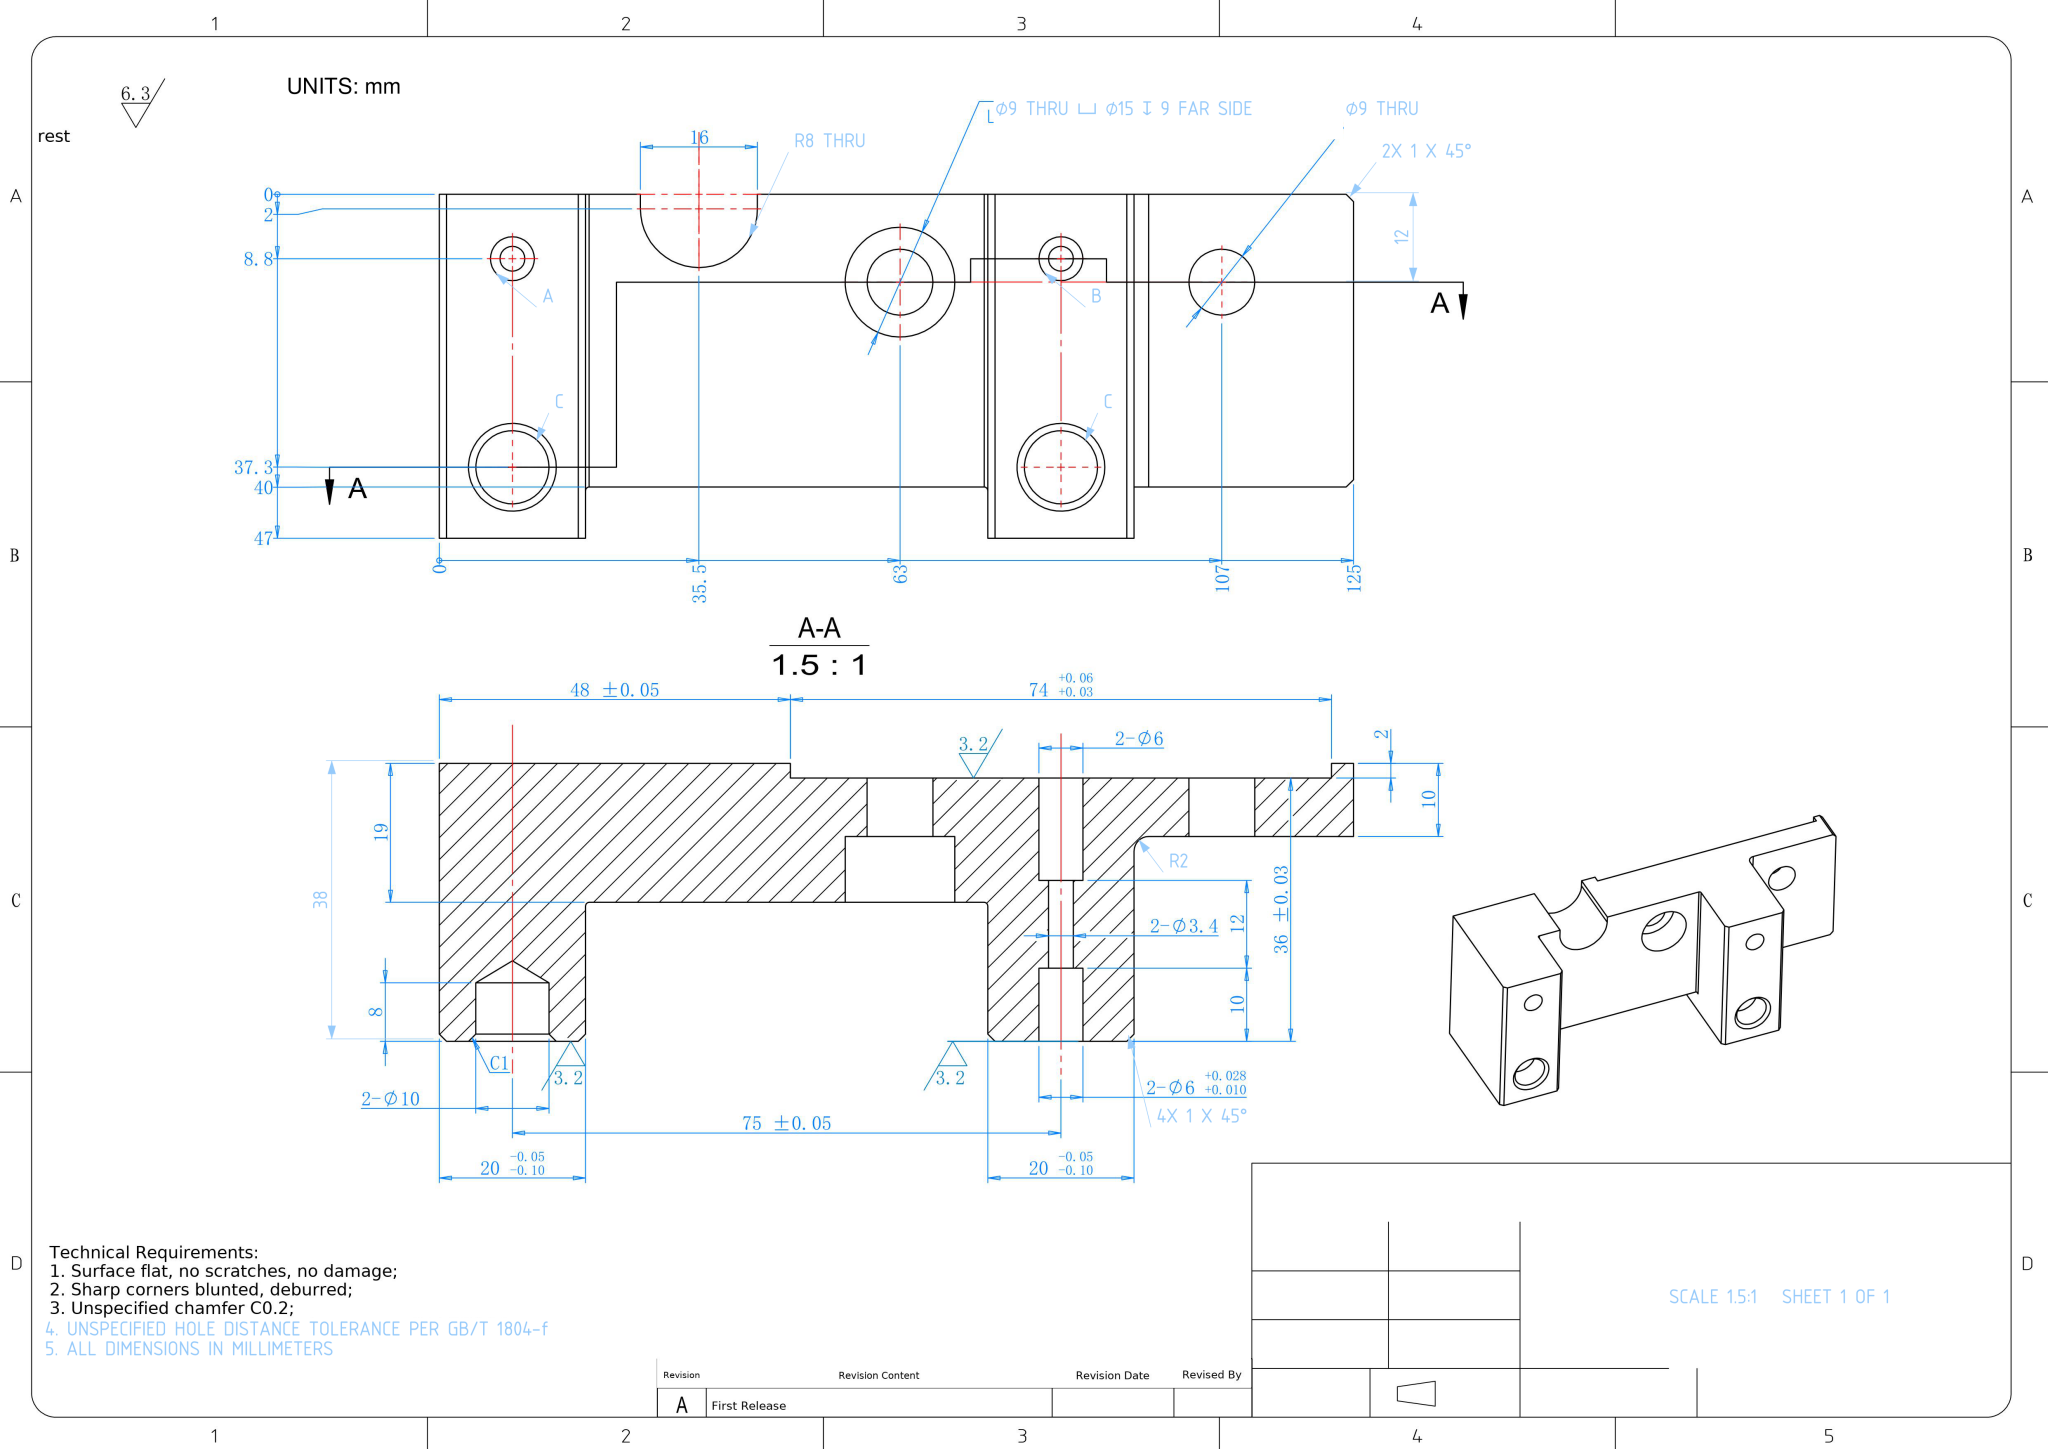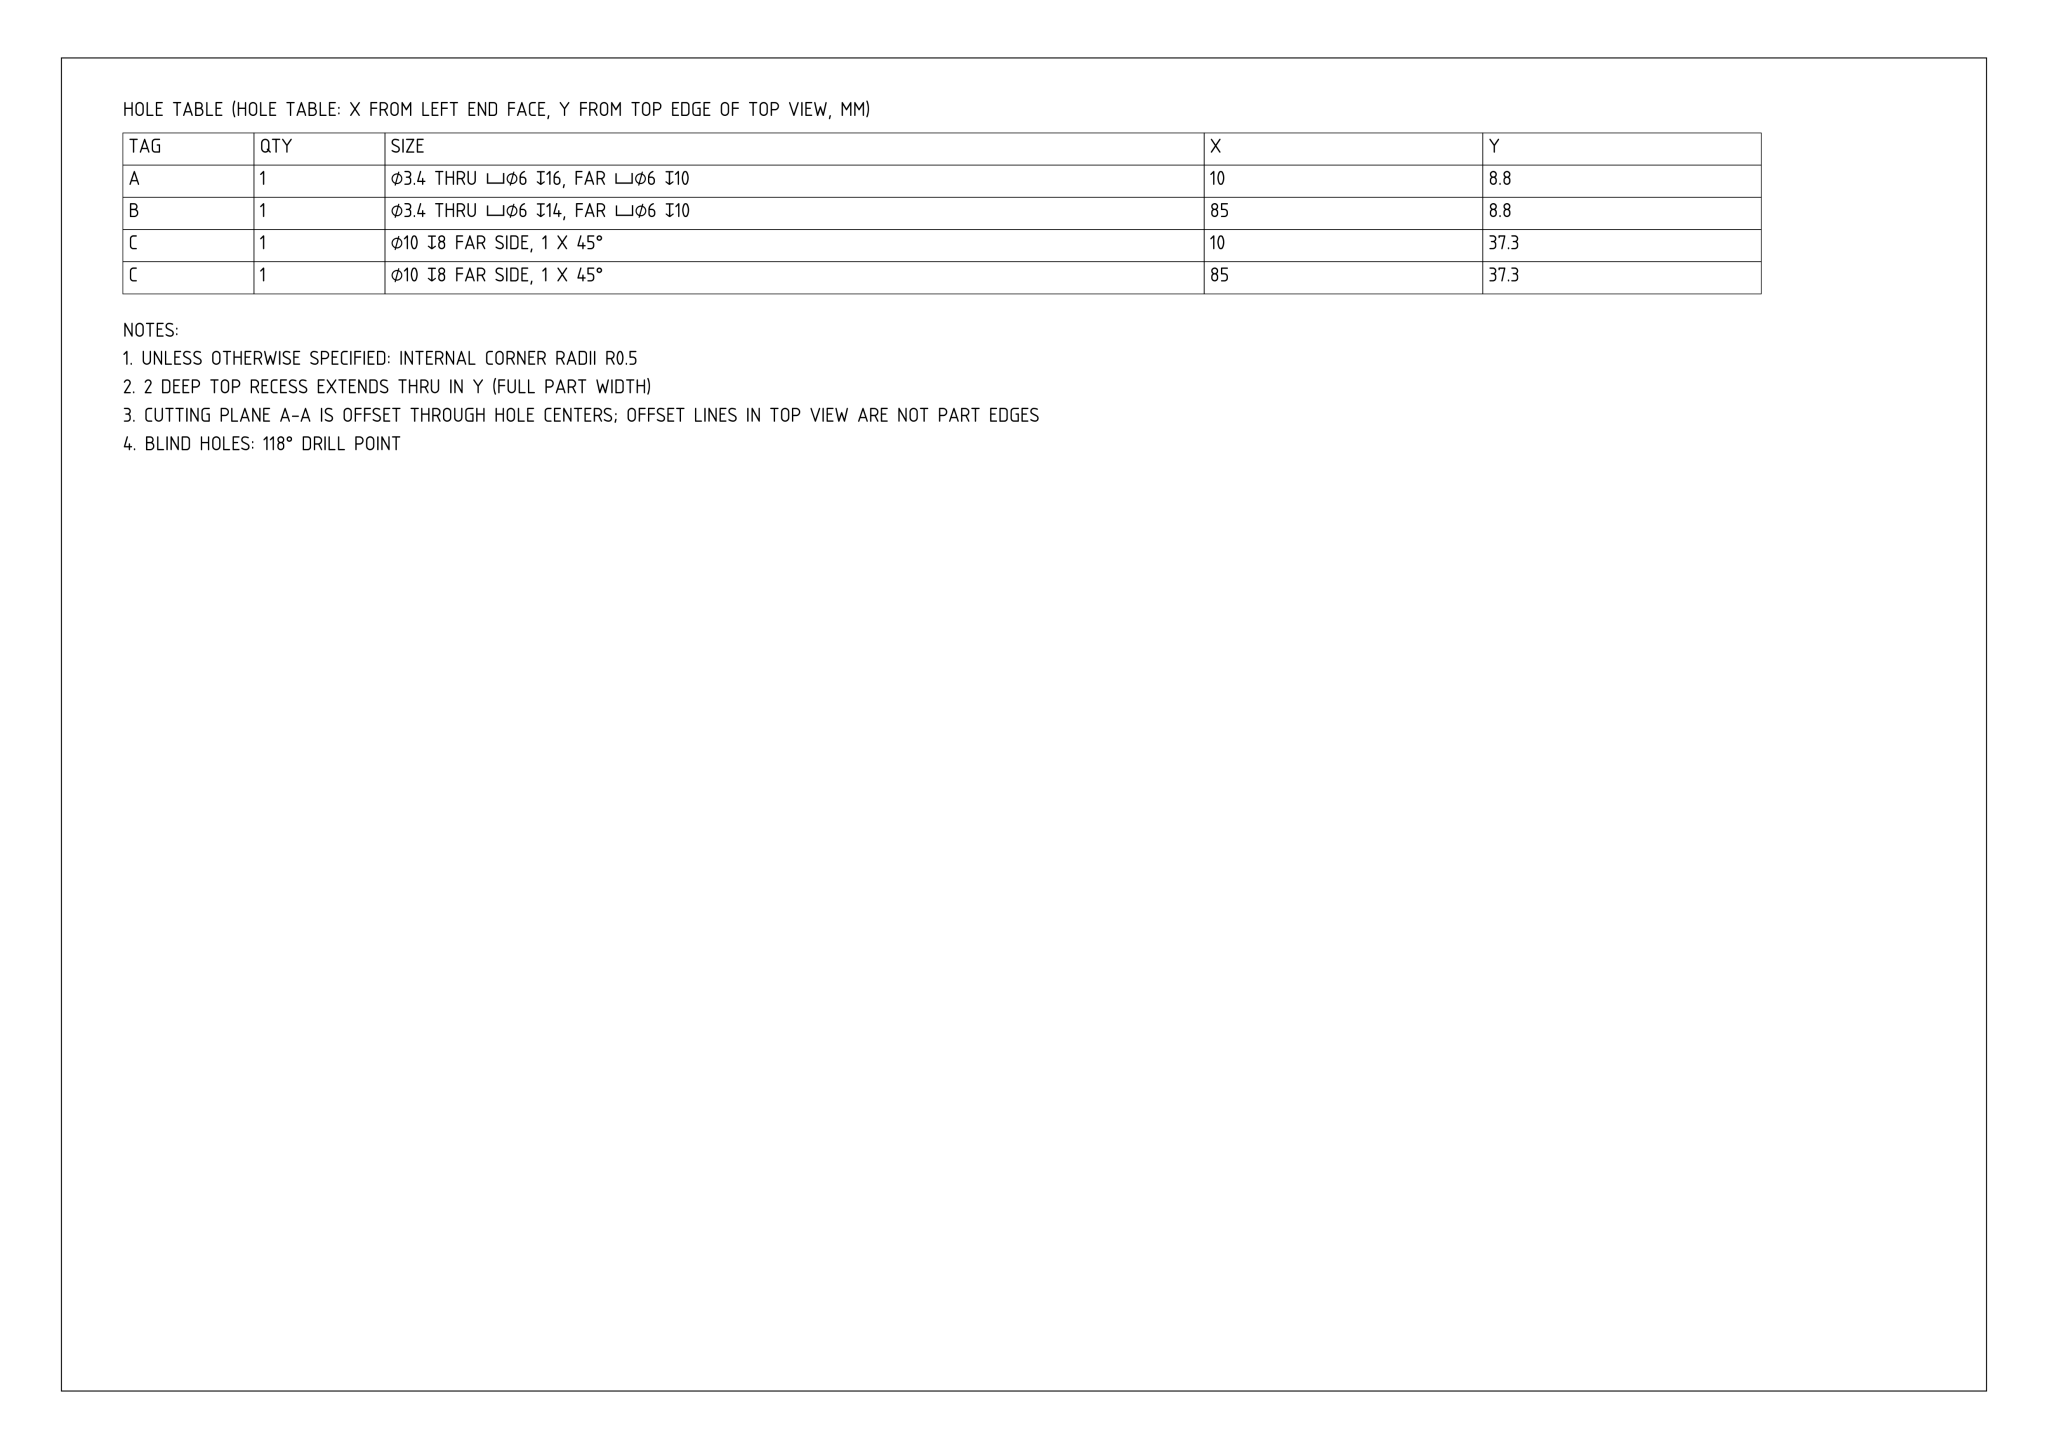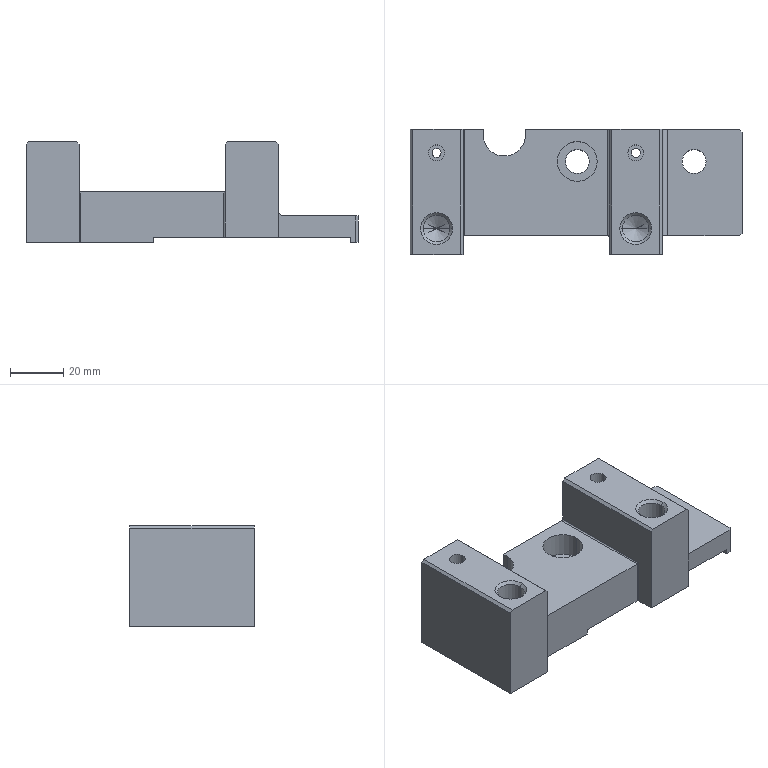Part | NX | mm | 1 solid | 69 faces | box 125 x 47 x 38 mm | volume 110771 mm3 | plane 33 | cylinder 28 | cone 8 | commonest cylinder face diameters 6 x8 9 x4 10 x4 3.4 x4 1 x4 15 x2 16 x1 4 x1